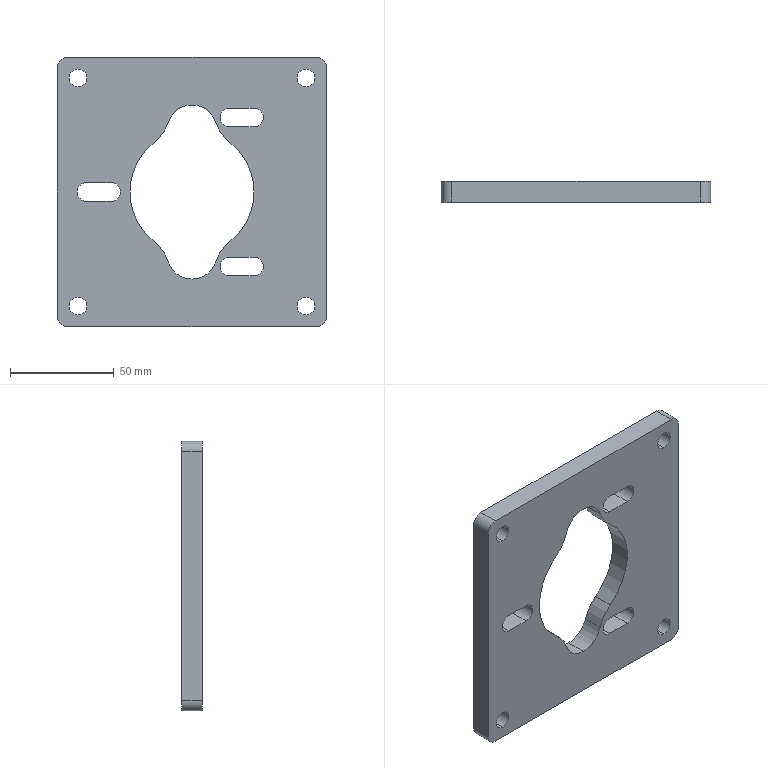Component | SolidWorks | Assembly4.1-1_UltrasonicConnectionBlock.1-1 | 1 solid | 39 faces | box 130 x 10 x 130 mm | volume 127827 mm3 | cylinder 27 | plane 12 | commonest cylinder face diameters 8.5 x8 9 x6 10 x4 40 x4 24 x3 60 x2
build123d program:
from build123d import *

# Parameters (mm, degrees)
SKETCH1_R           = 4.25
BOSS_EXTRUDE1_DEPTH = 10


with BuildPart() as part:
    # Sketch1 → Boss-Extrude1 (new body)
    with BuildSketch(Plane.XY):
        with BuildLine():
            Line((-60, 65), (60, 65))
            ThreePointArc((60, 65), (63.536, 63.536), (65, 60))
            Line((65, 60), (65, -60))
            ThreePointArc((65, -60), (63.536, -63.536), (60, -65))
            Line((60, -65), (-60, -65))
            ThreePointArc((-60, -65), (-63.536, -63.536), (-65, -60))
            Line((-65, -60), (-65, 60))
            ThreePointArc((-65, 60), (-63.536, 63.536), (-60, 65))
        make_face()
        with Locations((-55, 55)):
            Circle(SKETCH1_R, mode=Mode.SUBTRACT)
        with Locations((55, 55)):
            Circle(SKETCH1_R, mode=Mode.SUBTRACT)
        with Locations((55, -55)):
            Circle(SKETCH1_R, mode=Mode.SUBTRACT)
        with Locations((-55, -55)):
            Circle(SKETCH1_R, mode=Mode.SUBTRACT)
        with BuildLine():
            Line((4.5, -39), (4.5, -51))
            ThreePointArc((4.5, -51), (0, -55.5), (-4.5, -51))
            Line((-4.5, -51), (-4.5, -39))
            ThreePointArc((-4.5, -39), (0, -34.5), (4.5, -39))
        make_face(mode=Mode.SUBTRACT)
        with BuildLine():
            Line((-31.5, 30), (-31.5, 18))
            ThreePointArc((-31.5, 18), (-36, 13.5), (-40.5, 18))
            Line((-40.5, 18), (-40.5, 30))
            ThreePointArc((-40.5, 30), (-36, 34.5), (-31.5, 30))
        make_face(mode=Mode.SUBTRACT)
        with BuildLine():
            Line((40.5, 30), (40.5, 18))
            ThreePointArc((40.5, 18), (36, 13.5), (31.5, 18))
            Line((31.5, 18), (31.5, 30))
            ThreePointArc((31.5, 30), (36, 34.5), (40.5, 30))
        make_face(mode=Mode.SUBTRACT)
        with BuildLine():
            ThreePointArc((-23.76, -18.316), (0, -30), (23.76, -18.316))
            ThreePointArc((23.76, -18.316), (28.153, -14.126), (33.6, -11.447))
            ThreePointArc((33.6, -11.447), (42, 0), (33.6, 11.447))
            ThreePointArc((33.6, 11.447), (28.153, 14.126), (23.76, 18.316))
            ThreePointArc((23.76, 18.316), (0, 30), (-23.76, 18.316))
            ThreePointArc((-23.76, 18.316), (-28.153, 14.126), (-33.6, 11.447))
            ThreePointArc((-33.6, 11.447), (-42, 0), (-33.6, -11.447))
            ThreePointArc((-33.6, -11.447), (-28.153, -14.126), (-23.76, -18.316))
        make_face(mode=Mode.SUBTRACT)
    extrude(amount=BOSS_EXTRUDE1_DEPTH)


solid = part.part

# Placed as in the assembly
solid = solid.moved(Location((0, -47.5, -0.4), (90, 0, -90)))